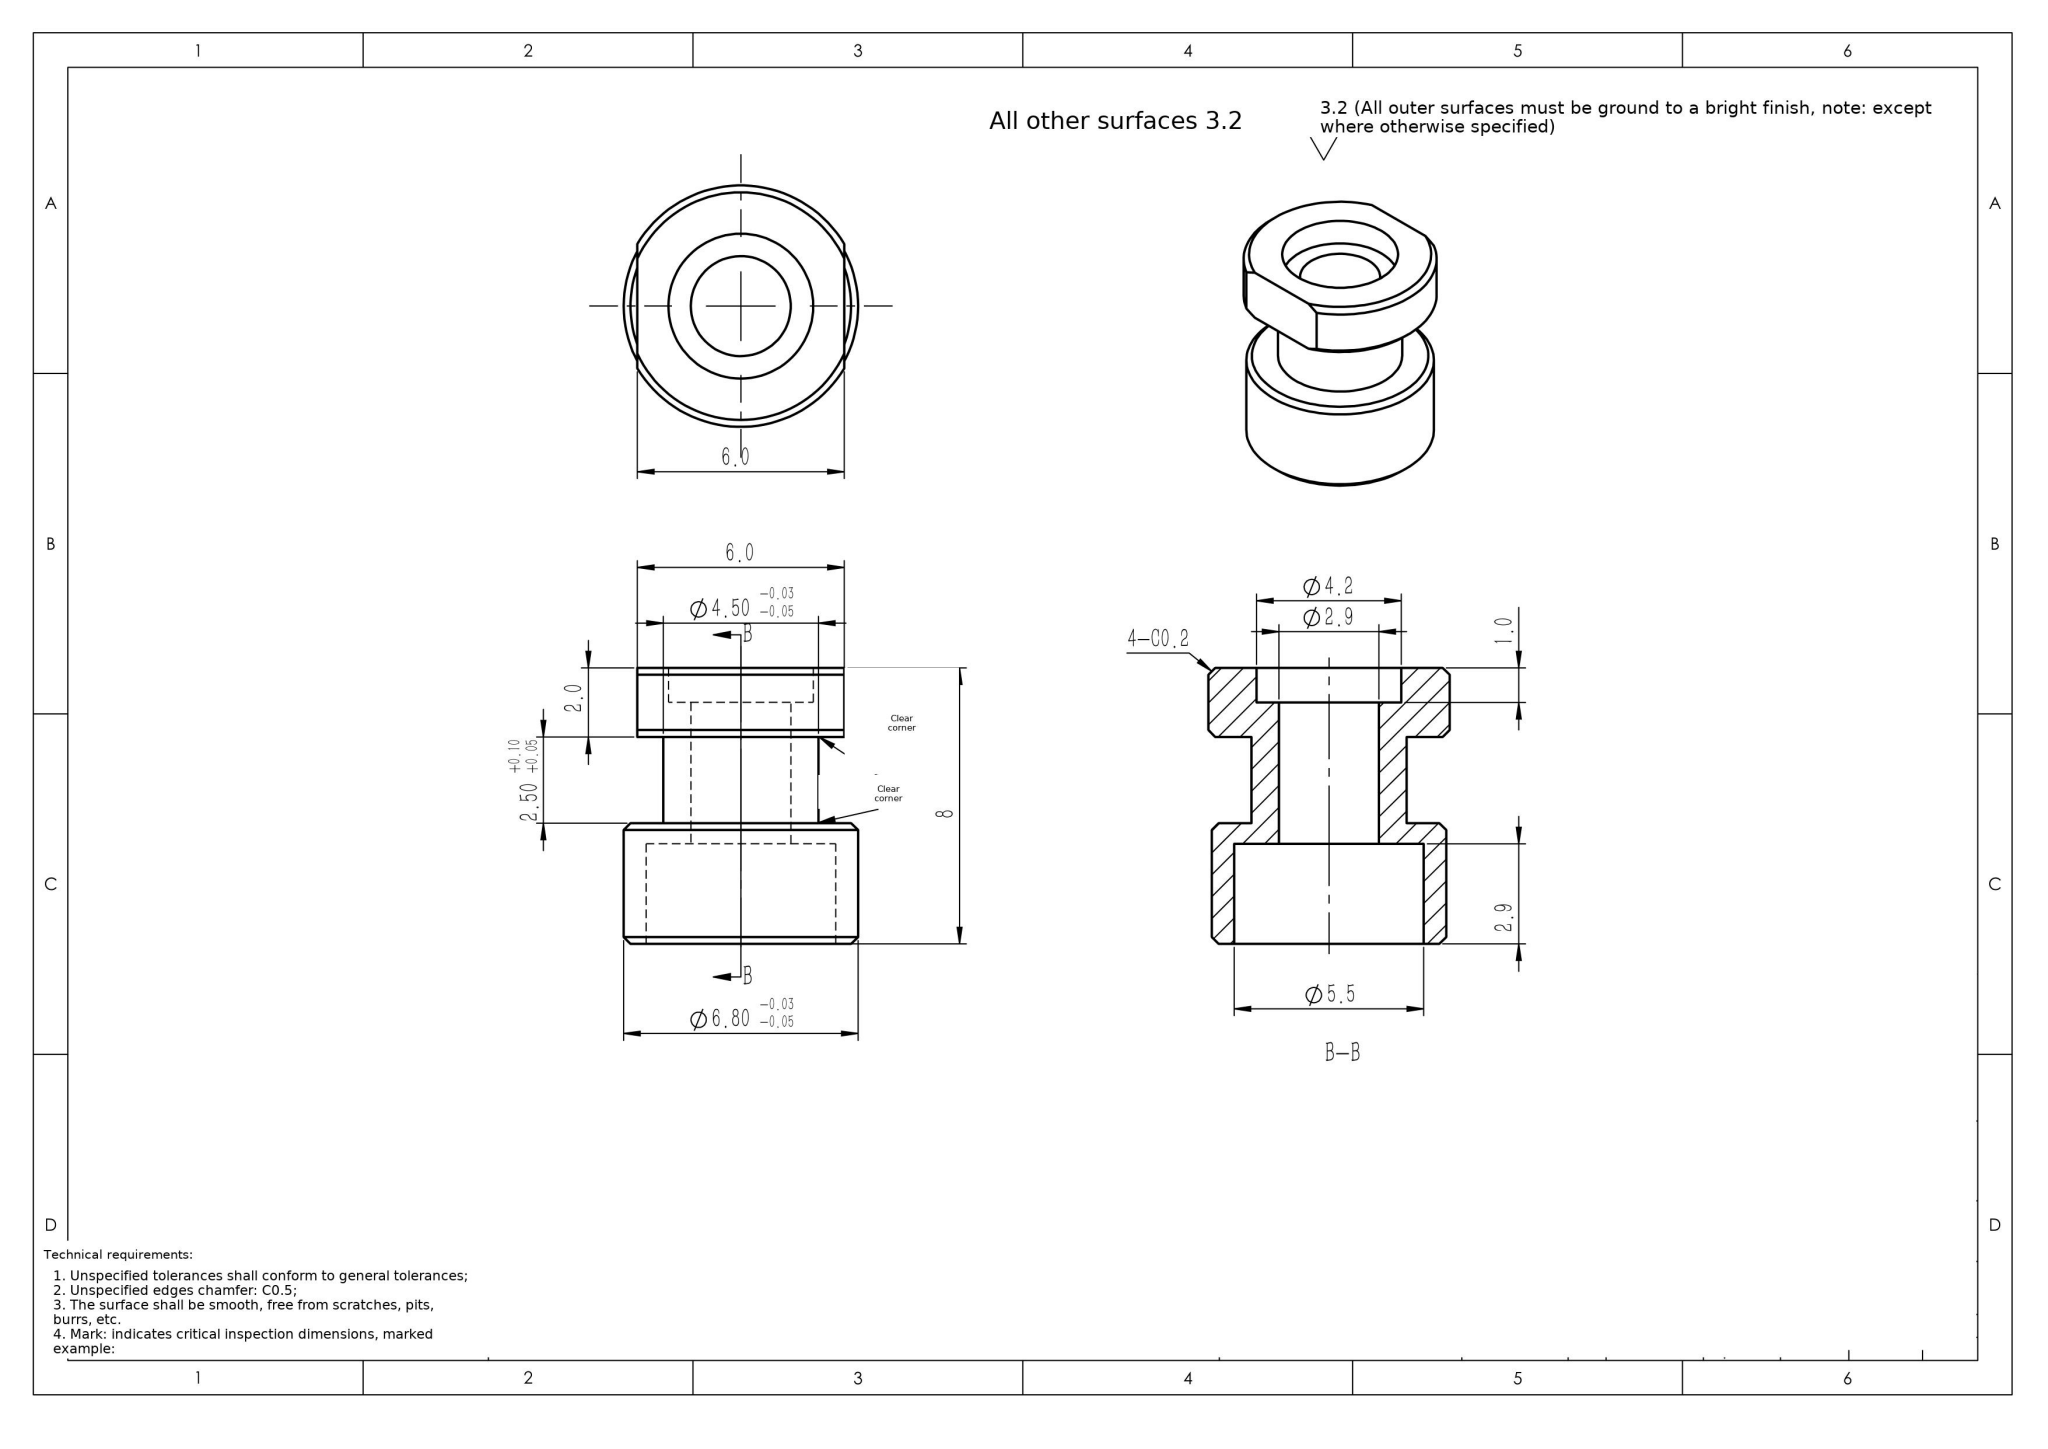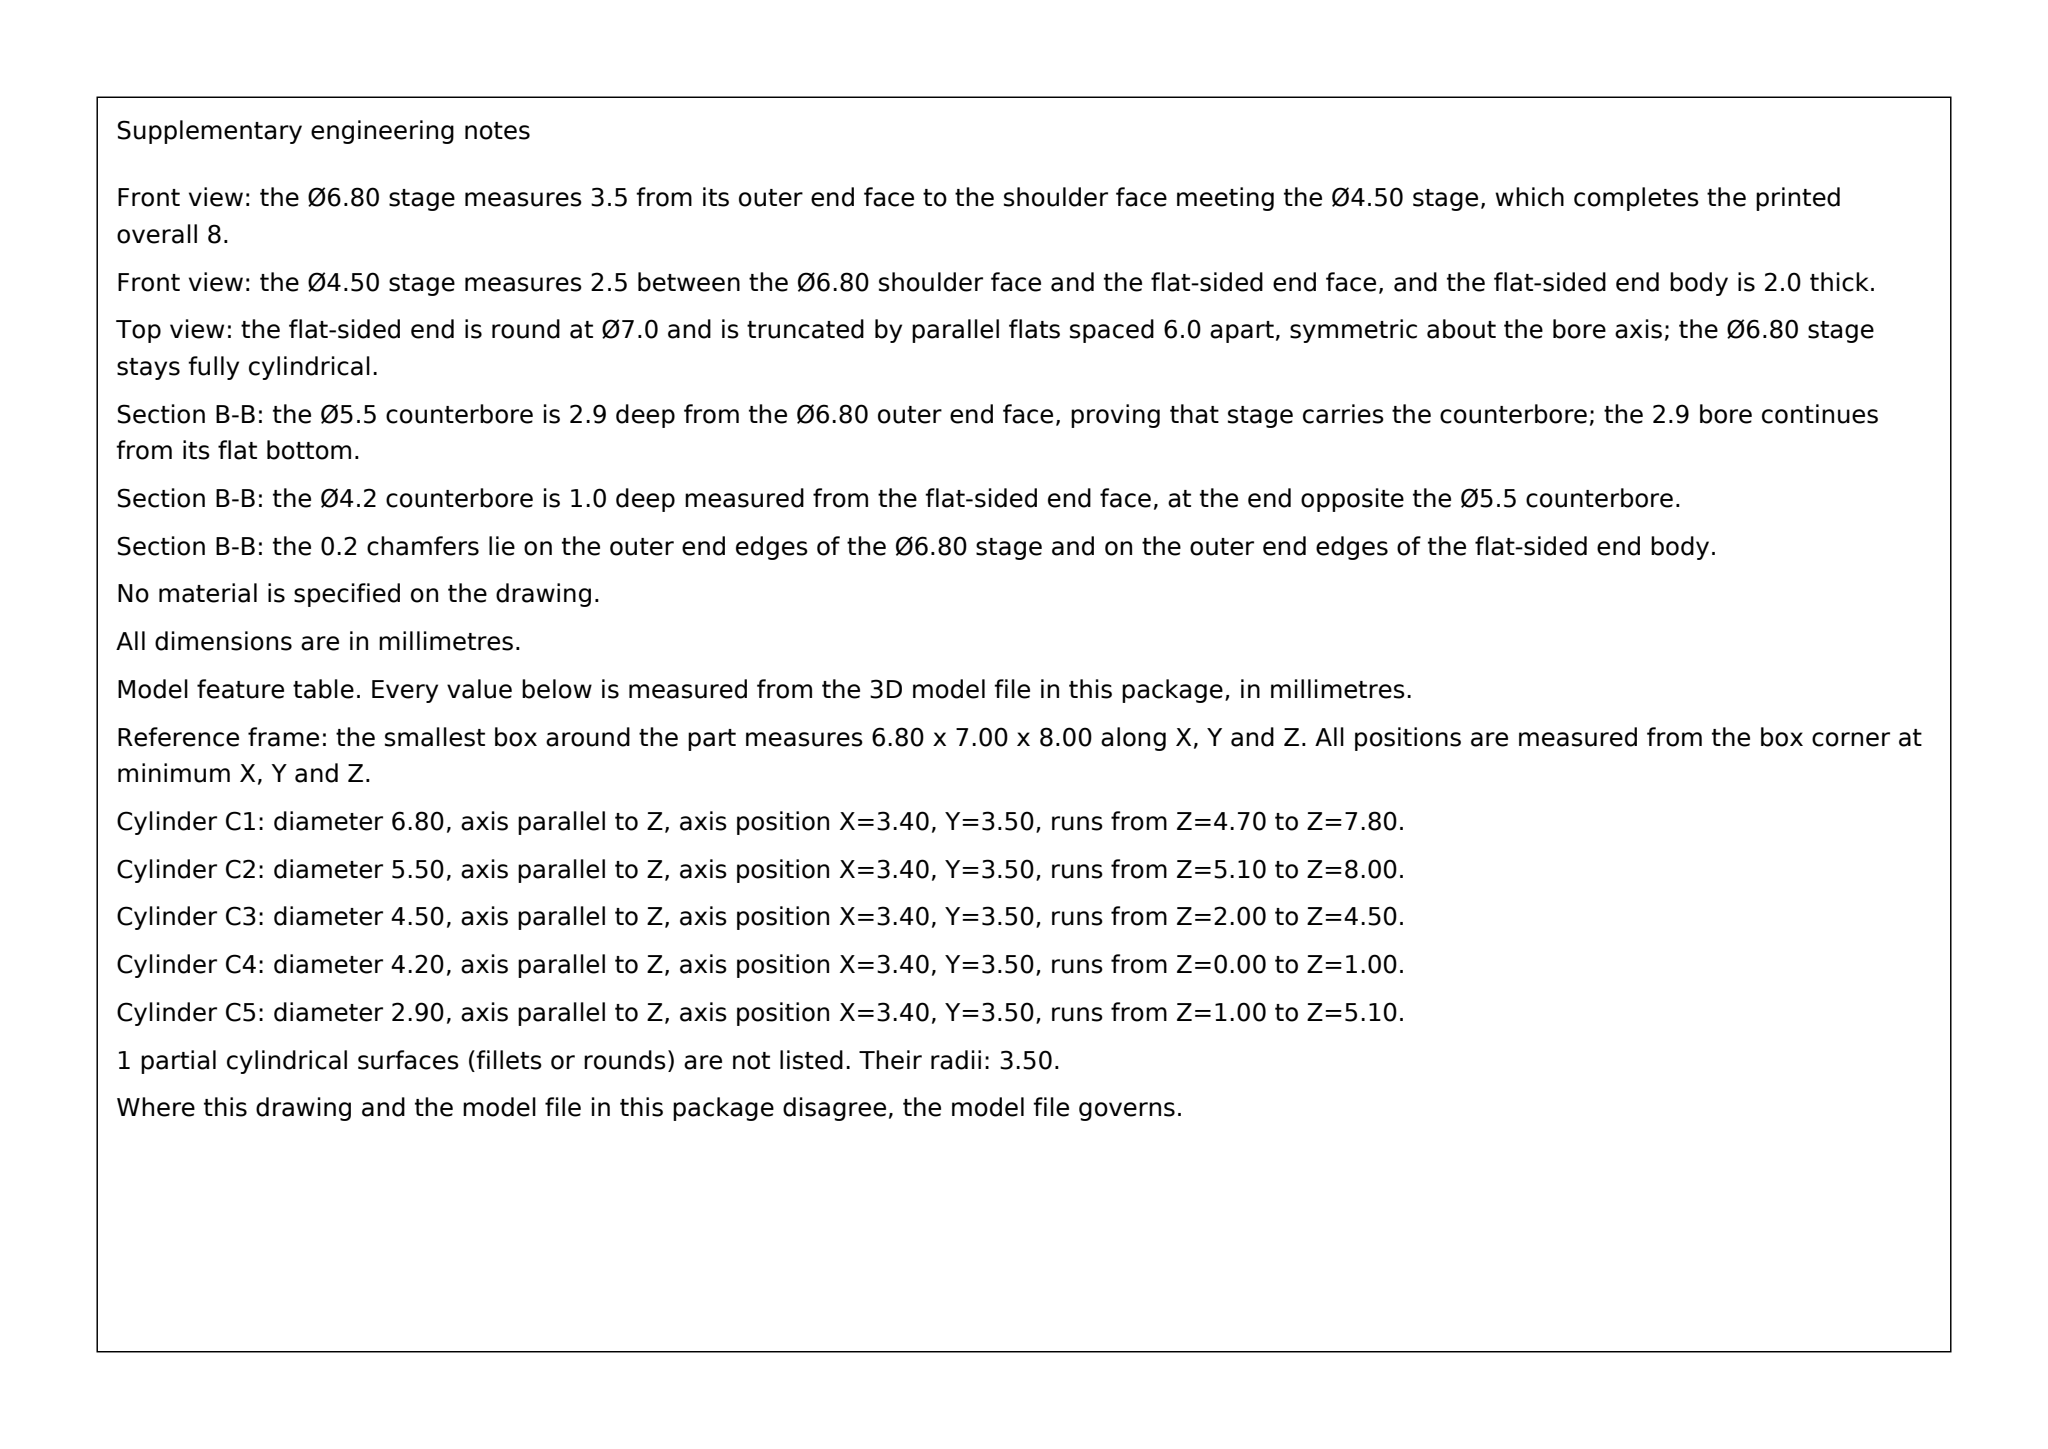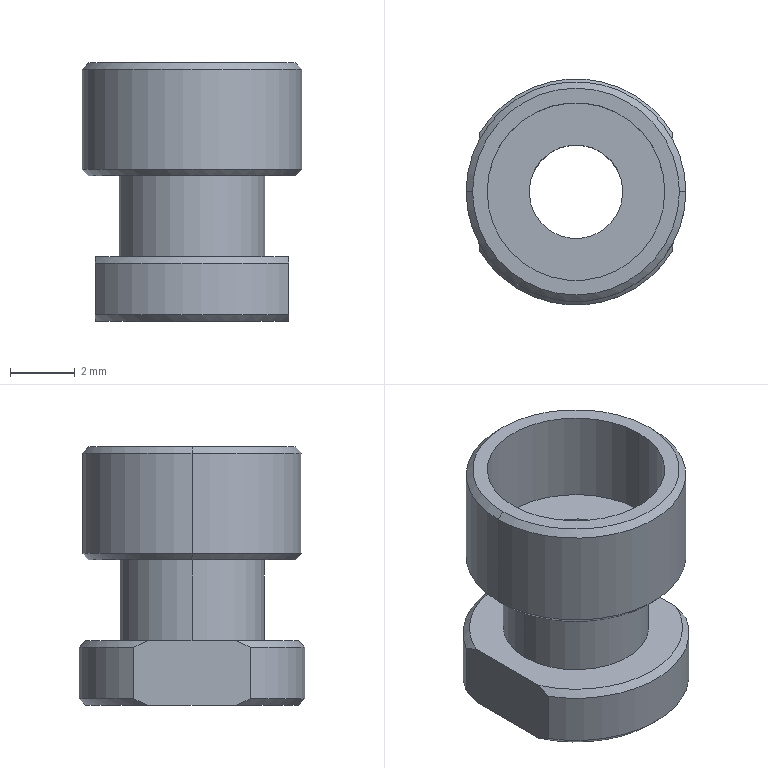Part | SolidWorks | mm | 1 solid | 28 faces | box 6.8 x 7 x 8 mm | volume 128 mm3 | cylinder 12 | cone 8 | plane 8 | commonest cylinder face diameters 4.2 x2 5.5 x2 4.5 x2 6.8 x2 2.9 x2 7 x2
Drawing notes:
Ø7.0 FLANGE W/ 2 FLATS 6.0 APART, 2.0 THK - NOT Ø6.80 BOSS | from the solid: Convex arc dia 7.0, axis z, z 0.2-1.8, arc 236 deg, with planes x=0.4 and x=6.4 (6.0 across flats), flange z 0.0-2.0; separate boss/shaft dia 6.8 z 4.7-7.8
build123d program:
from build123d import *

# Parameters (mm, degrees)
SKETCH1_R                                         = 3.4
BOSS_EXTRUDE1_DEPTH                               = 3.5
SKETCH2_R                                         = 2.25
BOSS_EXTRUDE2_DEPTH                               = 2.5
SKETCH3_R                                         = 3.5
BOSS_EXTRUDE3_DEPTH                               = 2
M2_5_HEX_SOCKET_HEAD_CAP_SCREW_CBORE2_D           = 2.9
M2_5_HEX_SOCKET_HEAD_CAP_SCREW_CBORE2_DEPTH       = 11.5
M2_5_HEX_SOCKET_HEAD_CAP_SCREW_CBORE2_CBORE_D     = 5.5
M2_5_HEX_SOCKET_HEAD_CAP_SCREW_CBORE2_CBORE_DEPTH = 2.9
M2_5_HEX_SOCKET_HEAD_CAP_SCREW_CBORE2_TIP         = 0.8712
SKETCH8_R                                         = 2.1
CUT_EXTRUDE1_DEPTH                                = 1
SKETCH9_W                                         = 1
SKETCH9_H                                         = 3.606
CUT_EXTRUDE2_DEPTH                                = 2
CHAMFER1_SIZE                                     = 0.2


with BuildPart() as part:
    # Sketch1 → Boss-Extrude1 (new body)
    with BuildSketch(Plane.XY):
        Circle(SKETCH1_R)
    extrude(amount=BOSS_EXTRUDE1_DEPTH)

    # Sketch2 → Boss-Extrude2 (add)
    with BuildSketch(Plane(origin=(0, 0, 0), x_dir=(-1, 0, 0), z_dir=(0, 0, -1))):
        with Locations(Location((0, 0, 0), (0, 0, 180))):
            Circle(SKETCH2_R)
    extrude(amount=BOSS_EXTRUDE2_DEPTH)

    # Sketch3 → Boss-Extrude3 (add)
    with BuildSketch(Plane(origin=(0, 0, -2.5), x_dir=(-1, 0, 0), z_dir=(0, 0, -1))):
        Circle(SKETCH3_R)
    extrude(amount=BOSS_EXTRUDE3_DEPTH)

    # M2.5 Hex Socket Head Cap Screw CBORE2
    with Locations(Plane.XY.offset(3.5)):
        with Locations((0, 0)):
            CounterBoreHole(M2_5_HEX_SOCKET_HEAD_CAP_SCREW_CBORE2_D / 2, M2_5_HEX_SOCKET_HEAD_CAP_SCREW_CBORE2_CBORE_D / 2, M2_5_HEX_SOCKET_HEAD_CAP_SCREW_CBORE2_CBORE_DEPTH, depth=M2_5_HEX_SOCKET_HEAD_CAP_SCREW_CBORE2_DEPTH)
            with Locations((0, 0, -(M2_5_HEX_SOCKET_HEAD_CAP_SCREW_CBORE2_DEPTH + M2_5_HEX_SOCKET_HEAD_CAP_SCREW_CBORE2_TIP / 2))):  # 118° drill point
                Cone(0, M2_5_HEX_SOCKET_HEAD_CAP_SCREW_CBORE2_D / 2, M2_5_HEX_SOCKET_HEAD_CAP_SCREW_CBORE2_TIP, mode=Mode.SUBTRACT)

    # Sketch8 → Cut-Extrude1 (cut)
    with BuildSketch(Plane(origin=(0, 0, -4.5), x_dir=(-1, 0, 0), z_dir=(0, 0, -1))):
        Circle(SKETCH8_R)
    extrude(amount=-CUT_EXTRUDE1_DEPTH, mode=Mode.SUBTRACT)

    # Sketch9 → Cut-Extrude2 (cut)
    with BuildSketch(Plane(origin=(0, 0, -4.5), x_dir=(-1, 0, 0), z_dir=(0, 0, -1))):
        with Locations((3.5, 0)):
            Rectangle(SKETCH9_W, SKETCH9_H)
        with Locations((-3.5, 0)):
            Rectangle(SKETCH9_W, SKETCH9_H)
    extrude(amount=-CUT_EXTRUDE2_DEPTH, mode=Mode.SUBTRACT)

    # Chamfer1
    chamfer1_edges = [part.edges().sort_by_distance(p)[0] for p in [
        (-3.4, 0, 0),
        (-3.4, 0, 3.5),
        (0, -3.5, -2.5),
        (0, -3.5, -4.5),
        (0, 3.5, -2.5),
        (0, 3.5, -4.5),
    ]]
    chamfer(chamfer1_edges, length=CHAMFER1_SIZE)


solid = part.part
STEP:
#1=CARTESIAN_POINT('',(3.2,0.,3.5));
#2=VERTEX_POINT('',#1);
#3=CARTESIAN_POINT('',(-3.2,0.,3.5));
#4=VERTEX_POINT('',#3);
#5=CARTESIAN_POINT('',(0.,0.,3.5));
#6=DIRECTION('',(0.,0.,1.));
#7=DIRECTION('',(1.,0.,0.));
#8=AXIS2_PLACEMENT_3D('',#5,#6,#7);
#9=CIRCLE('',#8,3.2);
#10=EDGE_CURVE('',#2,#4,#9,.T.);
#11=ORIENTED_EDGE('',*,*,#10,.F.);
#12=CARTESIAN_POINT('',(3.4,0.,3.3));
#13=VERTEX_POINT('',#12);
#14=CARTESIAN_POINT('',(3.2,0.,3.5));
#15=DIRECTION('',(0.7071,0.,-0.7071));
#16=VECTOR('',#15,1000.);
#17=LINE('',#14,#16);
#18=EDGE_CURVE('',#2,#13,#17,.T.);
#19=ORIENTED_EDGE('',*,*,#18,.T.);
#20=CARTESIAN_POINT('',(-3.4,0.,3.3));
#21=VERTEX_POINT('',#20);
#22=CARTESIAN_POINT('',(0.,0.,3.3));
#23=DIRECTION('',(0.,0.,-1.));
#24=DIRECTION('',(1.,0.,0.));
#25=AXIS2_PLACEMENT_3D('',#22,#23,#24);
#26=CIRCLE('',#25,3.4);
#27=EDGE_CURVE('',#21,#13,#26,.T.);
#28=ORIENTED_EDGE('',*,*,#27,.F.);
#29=CARTESIAN_POINT('',(-3.2,0.,3.5));
#30=DIRECTION('',(-0.7071,0.,-0.7071));
#31=VECTOR('',#30,1000.);
#32=LINE('',#29,#31);
#33=EDGE_CURVE('',#4,#21,#32,.T.);
#34=ORIENTED_EDGE('',*,*,#33,.F.);
#35=EDGE_LOOP('',(#11,#19,#28,#34));
#36=FACE_OUTER_BOUND('',#35,.T.);
#37=CARTESIAN_POINT('',(0.,0.,3.5));
#38=DIRECTION('',(0.,0.,-1.));
#39=DIRECTION('',(-1.,0.,0.));
#40=AXIS2_PLACEMENT_3D('',#37,#38,#39);
#41=CONICAL_SURFACE('',#40,3.2,0.7854);
#42=ADVANCED_FACE('',(#36),#41,.T.);
#43=CARTESIAN_POINT('',(-3.2,0.,0.));
#44=VERTEX_POINT('',#43);
#45=CARTESIAN_POINT('',(3.2,0.,0.));
#46=VERTEX_POINT('',#45);
#47=CARTESIAN_POINT('',(0.,0.,0.));
#48=DIRECTION('',(0.,0.,-1.));
#49=DIRECTION('',(1.,0.,0.));
#50=AXIS2_PLACEMENT_3D('',#47,#48,#49);
#51=CIRCLE('',#50,3.2);
#52=EDGE_CURVE('',#44,#46,#51,.T.);
#53=ORIENTED_EDGE('',*,*,#52,.F.);
#54=CARTESIAN_POINT('',(-3.4,0.,0.2));
#55=VERTEX_POINT('',#54);
#56=CARTESIAN_POINT('',(-3.4,0.,0.2));
#57=DIRECTION('',(-0.7071,0.,0.7071));
#58=VECTOR('',#57,1000.);
#59=LINE('',#56,#58);
#60=EDGE_CURVE('',#44,#55,#59,.T.);
#61=ORIENTED_EDGE('',*,*,#60,.T.);
#62=CARTESIAN_POINT('',(3.4,0.,0.2));
#63=VERTEX_POINT('',#62);
#64=CARTESIAN_POINT('',(0.,0.,0.2));
#65=DIRECTION('',(0.,0.,1.));
#66=DIRECTION('',(1.,0.,0.));
#67=AXIS2_PLACEMENT_3D('',#64,#65,#66);
#68=CIRCLE('',#67,3.4);
#69=EDGE_CURVE('',#63,#55,#68,.T.);
#70=ORIENTED_EDGE('',*,*,#69,.F.);
#71=CARTESIAN_POINT('',(3.4,0.,0.2));
#72=DIRECTION('',(0.7071,0.,0.7071));
#73=VECTOR('',#72,1000.);
#74=LINE('',#71,#73);
#75=EDGE_CURVE('',#46,#63,#74,.T.);
#76=ORIENTED_EDGE('',*,*,#75,.F.);
#77=EDGE_LOOP('',(#53,#61,#70,#76));
#78=FACE_OUTER_BOUND('',#77,.T.);
#79=CARTESIAN_POINT('',(0.,0.,0.2));
#80=DIRECTION('',(0.,0.,1.));
#81=DIRECTION('',(1.,0.,0.));
#82=AXIS2_PLACEMENT_3D('',#79,#80,#81);
#83=CONICAL_SURFACE('',#82,3.4,0.7854);
#84=ADVANCED_FACE('',(#78),#83,.T.);
#85=CARTESIAN_POINT('',(2.1,0.,-3.5));
#86=VERTEX_POINT('',#85);
#87=CARTESIAN_POINT('',(-2.1,0.,-3.5));
#88=VERTEX_POINT('',#87);
#89=CARTESIAN_POINT('',(0.,0.,-3.5));
#90=DIRECTION('',(0.,0.,-1.));
#91=DIRECTION('',(-1.,0.,0.));
#92=AXIS2_PLACEMENT_3D('',#89,#90,#91);
#93=CIRCLE('',#92,2.1);
#94=EDGE_CURVE('',#86,#88,#93,.T.);
#95=ORIENTED_EDGE('',*,*,#94,.F.);
#96=CARTESIAN_POINT('',(2.1,0.,-4.5));
#97=VERTEX_POINT('',#96);
#98=CARTESIAN_POINT('',(2.1,0.,-3.5));
#99=DIRECTION('',(0.,0.,-1.));
#100=VECTOR('',#99,1000.);
#101=LINE('',#98,#100);
#102=EDGE_CURVE('',#86,#97,#101,.T.);
#103=ORIENTED_EDGE('',*,*,#102,.T.);
#104=CARTESIAN_POINT('',(-2.1,0.,-4.5));
#105=VERTEX_POINT('',#104);
#106=CARTESIAN_POINT('',(0.,0.,-4.5));
#107=DIRECTION('',(0.,0.,-1.));
#108=DIRECTION('',(-1.,0.,0.));
#109=AXIS2_PLACEMENT_3D('',#106,#107,#108);
#110=CIRCLE('',#109,2.1);
#111=EDGE_CURVE('',#97,#105,#110,.T.);
#112=ORIENTED_EDGE('',*,*,#111,.T.);
#113=CARTESIAN_POINT('',(-2.1,0.,-3.5));
#114=DIRECTION('',(0.,0.,-1.));
#115=VECTOR('',#114,1000.);
#116=LINE('',#113,#115);
#117=EDGE_CURVE('',#88,#105,#116,.T.);
#118=ORIENTED_EDGE('',*,*,#117,.F.);
#119=EDGE_LOOP('',(#95,#103,#112,#118));
#120=FACE_OUTER_BOUND('',#119,.T.);
#121=CARTESIAN_POINT('',(0.,0.,-3.5));
#122=DIRECTION('',(0.,0.,-1.));
#123=DIRECTION('',(-1.,0.,0.));
#124=AXIS2_PLACEMENT_3D('',#121,#122,#123);
#125=CYLINDRICAL_SURFACE('',#124,2.1);
#126=ADVANCED_FACE('',(#120),#125,.F.);
#127=CARTESIAN_POINT('',(-2.75,0.,0.6));
#128=VERTEX_POINT('',#127);
#129=CARTESIAN_POINT('',(2.75,0.,0.6));
#130=VERTEX_POINT('',#129);
#131=CARTESIAN_POINT('',(0.,0.,0.6));
#132=DIRECTION('',(0.,0.,1.));
#133=DIRECTION('',(1.,0.,0.));
#134=AXIS2_PLACEMENT_3D('',#131,#132,#133);
#135=CIRCLE('',#134,2.75);
#136=EDGE_CURVE('',#128,#130,#135,.T.);
#137=ORIENTED_EDGE('',*,*,#136,.F.);
#138=CARTESIAN_POINT('',(-2.75,0.,3.5));
#139=VERTEX_POINT('',#138);
#140=CARTESIAN_POINT('',(-2.75,0.,3.5));
#141=DIRECTION('',(0.,0.,1.));
#142=VECTOR('',#141,1000.);
#143=LINE('',#140,#142);
#144=EDGE_CURVE('',#128,#139,#143,.T.);
#145=ORIENTED_EDGE('',*,*,#144,.T.);
#146=CARTESIAN_POINT('',(2.75,0.,3.5));
#147=VERTEX_POINT('',#146);
#148=CARTESIAN_POINT('',(0.,0.,3.5));
#149=DIRECTION('',(0.,0.,1.));
#150=DIRECTION('',(1.,0.,0.));
#151=AXIS2_PLACEMENT_3D('',#148,#149,#150);
#152=CIRCLE('',#151,2.75);
#153=EDGE_CURVE('',#139,#147,#152,.T.);
#154=ORIENTED_EDGE('',*,*,#153,.T.);
#155=CARTESIAN_POINT('',(2.75,0.,3.5));
#156=DIRECTION('',(0.,0.,1.));
#157=VECTOR('',#156,1000.);
#158=LINE('',#155,#157);
#159=EDGE_CURVE('',#130,#147,#158,.T.);
#160=ORIENTED_EDGE('',*,*,#159,.F.);
#161=EDGE_LOOP('',(#137,#145,#154,#160));
#162=FACE_OUTER_BOUND('',#161,.T.);
#163=CARTESIAN_POINT('',(0.,0.,3.5));
#164=DIRECTION('',(0.,0.,1.));
#165=DIRECTION('',(1.,0.,0.));
#166=AXIS2_PLACEMENT_3D('',#163,#164,#165);
#167=CYLINDRICAL_SURFACE('',#166,2.75);
#168=ADVANCED_FACE('',(#162),#167,.F.);
#169=CARTESIAN_POINT('',(-2.25,0.,-2.5));
#170=VERTEX_POINT('',#169);
#171=CARTESIAN_POINT('',(2.25,0.,-2.5));
#172=VERTEX_POINT('',#171);
#173=CARTESIAN_POINT('',(0.,0.,-2.5));
#174=DIRECTION('',(0.,0.,-1.));
#175=DIRECTION('',(-1.,0.,0.));
#176=AXIS2_PLACEMENT_3D('',#173,#174,#175);
#177=CIRCLE('',#176,2.25);
#178=EDGE_CURVE('',#170,#172,#177,.T.);
#179=ORIENTED_EDGE('',*,*,#178,.F.);
#180=CARTESIAN_POINT('',(-2.25,0.,0.));
#181=VERTEX_POINT('',#180);
#182=CARTESIAN_POINT('',(-2.25,0.,-2.5));
#183=DIRECTION('',(0.,0.,1.));
#184=VECTOR('',#183,1000.);
#185=LINE('',#182,#184);
#186=EDGE_CURVE('',#170,#181,#185,.T.);
#187=ORIENTED_EDGE('',*,*,#186,.T.);
#188=CARTESIAN_POINT('',(2.25,0.,0.));
#189=VERTEX_POINT('',#188);
#190=CARTESIAN_POINT('',(0.,0.,0.));
#191=DIRECTION('',(0.,0.,-1.));
#192=DIRECTION('',(1.,0.,0.));
#193=AXIS2_PLACEMENT_3D('',#190,#191,#192);
#194=CIRCLE('',#193,2.25);
#195=EDGE_CURVE('',#181,#189,#194,.T.);
#196=ORIENTED_EDGE('',*,*,#195,.T.);
#197=CARTESIAN_POINT('',(2.25,0.,-2.5));
#198=DIRECTION('',(0.,0.,1.));
#199=VECTOR('',#198,1000.);
#200=LINE('',#197,#199);
#201=EDGE_CURVE('',#172,#189,#200,.T.);
#202=ORIENTED_EDGE('',*,*,#201,.F.);
#203=EDGE_LOOP('',(#179,#187,#196,#202));
#204=FACE_OUTER_BOUND('',#203,.T.);
#205=CARTESIAN_POINT('',(0.,0.,-2.5));
#206=DIRECTION('',(0.,0.,1.));
#207=DIRECTION('',(1.,0.,0.));
#208=AXIS2_PLACEMENT_3D('',#205,#206,#207);
#209=CYLINDRICAL_SURFACE('',#208,2.25);
#210=ADVANCED_FACE('',(#204),#209,.T.);
#211=ORIENTED_EDGE('',*,*,#27,.T.);
#212=CARTESIAN_POINT('',(3.4,0.,3.5));
#213=DIRECTION('',(0.,0.,-1.));
#214=VECTOR('',#213,1000.);
#215=LINE('',#212,#214);
#216=EDGE_CURVE('',#13,#63,#215,.T.);
#217=ORIENTED_EDGE('',*,*,#216,.T.);
#218=ORIENTED_EDGE('',*,*,#69,.T.);
#219=CARTESIAN_POINT('',(-3.4,0.,3.5));
#220=DIRECTION('',(0.,0.,-1.));
#221=VECTOR('',#220,1000.);
#222=LINE('',#219,#221);
#223=EDGE_CURVE('',#21,#55,#222,.T.);
#224=ORIENTED_EDGE('',*,*,#223,.F.);
#225=EDGE_LOOP('',(#211,#217,#218,#224));
#226=FACE_OUTER_BOUND('',#225,.T.);
#227=CARTESIAN_POINT('',(0.,0.,3.5));
#228=DIRECTION('',(0.,0.,-1.));
#229=DIRECTION('',(-1.,0.,0.));
#230=AXIS2_PLACEMENT_3D('',#227,#228,#229);
#231=CYLINDRICAL_SURFACE('',#230,3.4);
#232=ADVANCED_FACE('',(#226),#231,.T.);
#233=CARTESIAN_POINT('',(-1.45,0.,-3.5));
#234=VERTEX_POINT('',#233);
#235=CARTESIAN_POINT('',(1.45,0.,-3.5));
#236=VERTEX_POINT('',#235);
#237=CARTESIAN_POINT('',(0.,0.,-3.5));
#238=DIRECTION('',(0.,0.,1.));
#239=DIRECTION('',(-1.,0.,0.));
#240=AXIS2_PLACEMENT_3D('',#237,#238,#239);
#241=CIRCLE('',#240,1.45);
#242=EDGE_CURVE('',#234,#236,#241,.T.);
#243=ORIENTED_EDGE('',*,*,#242,.F.);
#244=CARTESIAN_POINT('',(-1.45,0.,0.6));
#245=VERTEX_POINT('',#244);
#246=CARTESIAN_POINT('',(-1.45,0.,3.5));
#247=DIRECTION('',(0.,0.,1.));
#248=VECTOR('',#247,1000.);
#249=LINE('',#246,#248);
#250=EDGE_CURVE('',#234,#245,#249,.T.);
#251=ORIENTED_EDGE('',*,*,#250,.T.);
#252=CARTESIAN_POINT('',(1.45,0.,0.6));
#253=VERTEX_POINT('',#252);
#254=CARTESIAN_POINT('',(0.,0.,0.6));
#255=DIRECTION('',(0.,0.,1.));
#256=DIRECTION('',(1.,0.,0.));
#257=AXIS2_PLACEMENT_3D('',#254,#255,#256);
#258=CIRCLE('',#257,1.45);
#259=EDGE_CURVE('',#245,#253,#258,.T.);
#260=ORIENTED_EDGE('',*,*,#259,.T.);
#261=CARTESIAN_POINT('',(1.45,0.,3.5));
#262=DIRECTION('',(0.,0.,1.));
#263=VECTOR('',#262,1000.);
#264=LINE('',#261,#263);
#265=EDGE_CURVE('',#236,#253,#264,.T.);
#266=ORIENTED_EDGE('',*,*,#265,.F.);
#267=EDGE_LOOP('',(#243,#251,#260,#266));
#268=FACE_OUTER_BOUND('',#267,.T.);
#269=CARTESIAN_POINT('',(0.,0.,3.5));
#270=DIRECTION('',(0.,0.,1.));
#271=DIRECTION('',(1.,0.,0.));
#272=AXIS2_PLACEMENT_3D('',#269,#270,#271);
#273=CYLINDRICAL_SURFACE('',#272,1.45);
#274=ADVANCED_FACE('',(#268),#273,.F.);
#275=CARTESIAN_POINT('',(-3.,-1.803,-2.7));
#276=VERTEX_POINT('',#275);
#277=CARTESIAN_POINT('',(-3.,-1.803,-4.3));
#278=VERTEX_POINT('',#277);
#279=CARTESIAN_POINT('',(-3.,-1.803,1.242));
#280=DIRECTION('',(0.,0.,-1.));
#281=VECTOR('',#280,1000.);
#282=LINE('',#279,#281);
#283=EDGE_CURVE('',#276,#278,#282,.T.);
#284=ORIENTED_EDGE('',*,*,#283,.T.);
#285=CARTESIAN_POINT('',(3.,-1.803,-4.3));
#286=VERTEX_POINT('',#285);
#287=CARTESIAN_POINT('',(0.,0.,-4.3));
#288=DIRECTION('',(0.,0.,1.));
#289=DIRECTION('',(-1.,0.,0.));
#290=AXIS2_PLACEMENT_3D('',#287,#288,#289);
#291=CIRCLE('',#290,3.5);
#292=EDGE_CURVE('',#278,#286,#291,.T.);
#293=ORIENTED_EDGE('',*,*,#292,.T.);
#294=CARTESIAN_POINT('',(3.,-1.803,-2.7));
#295=VERTEX_POINT('',#294);
#296=CARTESIAN_POINT('',(3.,-1.803,1.242));
#297=DIRECTION('',(0.,0.,-1.));
#298=VECTOR('',#297,1000.);
#299=LINE('',#296,#298);
#300=EDGE_CURVE('',#295,#286,#299,.T.);
#301=ORIENTED_EDGE('',*,*,#300,.F.);
#302=CARTESIAN_POINT('',(0.,0.,-2.7));
#303=DIRECTION('',(0.,0.,-1.));
#304=DIRECTION('',(-1.,0.,0.));
#305=AXIS2_PLACEMENT_3D('',#302,#303,#304);
#306=CIRCLE('',#305,3.5);
#307=EDGE_CURVE('',#295,#276,#306,.T.);
#308=ORIENTED_EDGE('',*,*,#307,.T.);
#309=EDGE_LOOP('',(#284,#293,#301,#308));
#310=FACE_OUTER_BOUND('',#309,.T.);
#311=CARTESIAN_POINT('',(0.,0.,-4.5));
#312=DIRECTION('',(0.,0.,1.));
#313=DIRECTION('',(1.,0.,0.));
#314=AXIS2_PLACEMENT_3D('',#311,#312,#313);
#315=CYLINDRICAL_SURFACE('',#314,3.5);
#316=ADVANCED_FACE('',(#310),#315,.T.);
#317=ORIENTED_EDGE('',*,*,#250,.F.);
#318=CARTESIAN_POINT('',(0.,0.,-3.5));
#319=DIRECTION('',(0.,0.,1.));
#320=DIRECTION('',(-1.,0.,0.));
#321=AXIS2_PLACEMENT_3D('',#318,#319,#320);
#322=CIRCLE('',#321,1.45);
#323=EDGE_CURVE('',#236,#234,#322,.T.);
#324=ORIENTED_EDGE('',*,*,#323,.F.);
#325=ORIENTED_EDGE('',*,*,#265,.T.);
#326=CARTESIAN_POINT('',(0.,0.,0.6));
#327=DIRECTION('',(0.,0.,1.));
#328=DIRECTION('',(1.,0.,0.));
#329=AXIS2_PLACEMENT_3D('',#326,#327,#328);
#330=CIRCLE('',#329,1.45);
#331=EDGE_CURVE('',#253,#245,#330,.T.);
#332=ORIENTED_EDGE('',*,*,#331,.T.);
#333=EDGE_LOOP('',(#317,#324,#325,#332));
#334=FACE_OUTER_BOUND('',#333,.T.);
#335=CARTESIAN_POINT('',(0.,0.,3.5));
#336=DIRECTION('',(0.,0.,1.));
#337=DIRECTION('',(1.,0.,0.));
#338=AXIS2_PLACEMENT_3D('',#335,#336,#337);
#339=CYLINDRICAL_SURFACE('',#338,1.45);
#340=ADVANCED_FACE('',(#334),#339,.F.);
#341=ORIENTED_EDGE('',*,*,#216,.F.);
#342=CARTESIAN_POINT('',(0.,0.,3.3));
#343=DIRECTION('',(0.,0.,-1.));
#344=DIRECTION('',(1.,0.,0.));
#345=AXIS2_PLACEMENT_3D('',#342,#343,#344);
#346=CIRCLE('',#345,3.4);
#347=EDGE_CURVE('',#13,#21,#346,.T.);
#348=ORIENTED_EDGE('',*,*,#347,.T.);
#349=ORIENTED_EDGE('',*,*,#223,.T.);
#350=CARTESIAN_POINT('',(0.,0.,0.2));
#351=DIRECTION('',(0.,0.,1.));
#352=DIRECTION('',(1.,0.,0.));
#353=AXIS2_PLACEMENT_3D('',#350,#351,#352);
#354=CIRCLE('',#353,3.4);
#355=EDGE_CURVE('',#55,#63,#354,.T.);
#356=ORIENTED_EDGE('',*,*,#355,.T.);
#357=EDGE_LOOP('',(#341,#348,#349,#356));
#358=FACE_OUTER_BOUND('',#357,.T.);
#359=CARTESIAN_POINT('',(0.,0.,3.5));
#360=DIRECTION('',(0.,0.,-1.));
#361=DIRECTION('',(-1.,0.,0.));
#362=AXIS2_PLACEMENT_3D('',#359,#360,#361);
#363=CYLINDRICAL_SURFACE('',#362,3.4);
#364=ADVANCED_FACE('',(#358),#363,.T.);
#365=CARTESIAN_POINT('',(0.,0.,3.5));
#366=DIRECTION('',(0.,0.,1.));
#367=DIRECTION('',(1.,0.,0.));
#368=AXIS2_PLACEMENT_3D('',#365,#366,#367);
#369=CIRCLE('',#368,3.2);
#370=EDGE_CURVE('',#4,#2,#369,.T.);
#371=ORIENTED_EDGE('',*,*,#370,.T.);
#372=ORIENTED_EDGE('',*,*,#10,.T.);
#373=EDGE_LOOP('',(#371,#372));
#374=FACE_OUTER_BOUND('',#373,.T.);
#375=CARTESIAN_POINT('',(0.,0.,3.5));
#376=DIRECTION('',(0.,0.,1.));
#377=DIRECTION('',(1.,0.,0.));
#378=AXIS2_PLACEMENT_3D('',#375,#376,#377);
#379=CIRCLE('',#378,2.75);
#380=EDGE_CURVE('',#147,#139,#379,.T.);
#381=ORIENTED_EDGE('',*,*,#380,.F.);
#382=ORIENTED_EDGE('',*,*,#153,.F.);
#383=EDGE_LOOP('',(#381,#382));
#384=FACE_BOUND('',#383,.T.);
#385=CARTESIAN_POINT('',(0.,0.,3.5));
#386=DIRECTION('',(0.,0.,1.));
#387=DIRECTION('',(1.,0.,0.));
#388=AXIS2_PLACEMENT_3D('',#385,#386,#387);
#389=PLANE('',#388);
#390=ADVANCED_FACE('',(#374,#384),#389,.T.);
#391=CARTESIAN_POINT('',(0.,0.,0.));
#392=DIRECTION('',(0.,0.,-1.));
#393=DIRECTION('',(1.,0.,0.));
#394=AXIS2_PLACEMENT_3D('',#391,#392,#393);
#395=CIRCLE('',#394,3.2);
#396=EDGE_CURVE('',#46,#44,#395,.T.);
#397=ORIENTED_EDGE('',*,*,#396,.T.);
#398=ORIENTED_EDGE('',*,*,#52,.T.);
#399=EDGE_LOOP('',(#397,#398));
#400=FACE_OUTER_BOUND('',#399,.T.);
#401=CARTESIAN_POINT('',(0.,0.,0.));
#402=DIRECTION('',(0.,0.,-1.));
#403=DIRECTION('',(1.,0.,0.));
#404=AXIS2_PLACEMENT_3D('',#401,#402,#403);
#405=CIRCLE('',#404,2.25);
#406=EDGE_CURVE('',#189,#181,#405,.T.);
#407=ORIENTED_EDGE('',*,*,#406,.F.);
#408=ORIENTED_EDGE('',*,*,#195,.F.);
#409=EDGE_LOOP('',(#407,#408));
#410=FACE_BOUND('',#409,.T.);
#411=CARTESIAN_POINT('',(0.,0.,0.));
#412=DIRECTION('',(0.,0.,1.));
#413=DIRECTION('',(1.,0.,0.));
#414=AXIS2_PLACEMENT_3D('',#411,#412,#413);
#415=PLANE('',#414);
#416=ADVANCED_FACE('',(#400,#410),#415,.F.);
#417=ORIENTED_EDGE('',*,*,#186,.F.);
#418=CARTESIAN_POINT('',(0.,0.,-2.5));
#419=DIRECTION('',(0.,0.,-1.));
#420=DIRECTION('',(-1.,0.,0.));
#421=AXIS2_PLACEMENT_3D('',#418,#419,#420);
#422=CIRCLE('',#421,2.25);
#423=EDGE_CURVE('',#172,#170,#422,.T.);
#424=ORIENTED_EDGE('',*,*,#423,.F.);
#425=ORIENTED_EDGE('',*,*,#201,.T.);
#426=ORIENTED_EDGE('',*,*,#406,.T.);
#427=EDGE_LOOP('',(#417,#424,#425,#426));
#428=FACE_OUTER_BOUND('',#427,.T.);
#429=CARTESIAN_POINT('',(0.,0.,-2.5));
#430=DIRECTION('',(0.,0.,1.));
#431=DIRECTION('',(1.,0.,0.));
#432=AXIS2_PLACEMENT_3D('',#429,#430,#431);
#433=CYLINDRICAL_SURFACE('',#432,2.25);
#434=ADVANCED_FACE('',(#428),#433,.T.);
#435=CARTESIAN_POINT('',(3.,1.803,-2.7));
#436=VERTEX_POINT('',#435);
#437=CARTESIAN_POINT('',(3.,1.803,-4.3));
#438=VERTEX_POINT('',#437);
#439=CARTESIAN_POINT('',(3.,1.803,1.242));
#440=DIRECTION('',(0.,0.,-1.));
#441=VECTOR('',#440,1000.);
#442=LINE('',#439,#441);
#443=EDGE_CURVE('',#436,#438,#442,.T.);
#444=ORIENTED_EDGE('',*,*,#443,.T.);
#445=CARTESIAN_POINT('',(-3.,1.803,-4.3));
#446=VERTEX_POINT('',#445);
#447=CARTESIAN_POINT('',(0.,0.,-4.3));
#448=DIRECTION('',(0.,0.,1.));
#449=DIRECTION('',(-1.,-0.,0.));
#450=AXIS2_PLACEMENT_3D('',#447,#448,#449);
#451=CIRCLE('',#450,3.5);
#452=EDGE_CURVE('',#438,#446,#451,.T.);
#453=ORIENTED_EDGE('',*,*,#452,.T.);
#454=CARTESIAN_POINT('',(-3.,1.803,-2.7));
#455=VERTEX_POINT('',#454);
#456=CARTESIAN_POINT('',(-3.,1.803,1.242));
#457=DIRECTION('',(0.,0.,-1.));
#458=VECTOR('',#457,1000.);
#459=LINE('',#456,#458);
#460=EDGE_CURVE('',#455,#446,#459,.T.);
#461=ORIENTED_EDGE('',*,*,#460,.F.);
#462=CARTESIAN_POINT('',(0.,0.,-2.7));
#463=DIRECTION('',(0.,0.,-1.));
#464=DIRECTION('',(-1.,0.,0.));
#465=AXIS2_PLACEMENT_3D('',#462,#463,#464);
#466=CIRCLE('',#465,3.5);
#467=EDGE_CURVE('',#455,#436,#466,.T.);
#468=ORIENTED_EDGE('',*,*,#467,.T.);
#469=EDGE_LOOP('',(#444,#453,#461,#468));
#470=FACE_OUTER_BOUND('',#469,.T.);
#471=CARTESIAN_POINT('',(0.,0.,-4.5));
#472=DIRECTION('',(0.,0.,1.));
#473=DIRECTION('',(1.,0.,0.));
#474=AXIS2_PLACEMENT_3D('',#471,#472,#473);
#475=CYLINDRICAL_SURFACE('',#474,3.5);
#476=ADVANCED_FACE('',(#470),#475,.T.);
#477=CARTESIAN_POINT('',(-3.,1.375,-4.5));
#478=VERTEX_POINT('',#477);
#479=CARTESIAN_POINT('',(-3.,-1.375,-4.5));
#480=VERTEX_POINT('',#479);
#481=CARTESIAN_POINT('',(-3.,1.803,-4.5));
#482=DIRECTION('',(0.,-1.,0.));
#483=VECTOR('',#482,1000.);
#484=LINE('',#481,#483);
#485=EDGE_CURVE('',#478,#480,#484,.T.);
#486=ORIENTED_EDGE('',*,*,#485,.F.);
#487=CARTESIAN_POINT('',(3.,1.375,-4.5));
#488=VERTEX_POINT('',#487);
#489=CARTESIAN_POINT('',(0.,0.,-4.5));
#490=DIRECTION('',(0.,0.,-1.));
#491=DIRECTION('',(-1.,0.,0.));
#492=AXIS2_PLACEMENT_3D('',#489,#490,#491);
#493=CIRCLE('',#492,3.3);
#494=EDGE_CURVE('',#478,#488,#493,.T.);
#495=ORIENTED_EDGE('',*,*,#494,.T.);
#496=CARTESIAN_POINT('',(3.,-1.375,-4.5));
#497=VERTEX_POINT('',#496);
#498=CARTESIAN_POINT('',(3.,-1.803,-4.5));
#499=DIRECTION('',(0.,1.,0.));
#500=VECTOR('',#499,1000.);
#501=LINE('',#498,#500);
#502=EDGE_CURVE('',#497,#488,#501,.T.);
#503=ORIENTED_EDGE('',*,*,#502,.F.);
#504=CARTESIAN_POINT('',(0.,0.,-4.5));
#505=DIRECTION('',(0.,0.,-1.));
#506=DIRECTION('',(-1.,0.,0.));
#507=AXIS2_PLACEMENT_3D('',#504,#505,#506);
#508=CIRCLE('',#507,3.3);
#509=EDGE_CURVE('',#497,#480,#508,.T.);
#510=ORIENTED_EDGE('',*,*,#509,.T.);
#511=EDGE_LOOP('',(#486,#495,#503,#510));
#512=FACE_OUTER_BOUND('',#511,.T.);
#513=CARTESIAN_POINT('',(0.,0.,-4.5));
#514=DIRECTION('',(0.,0.,-1.));
#515=DIRECTION('',(-1.,0.,0.));
#516=AXIS2_PLACEMENT_3D('',#513,#514,#515);
#517=CIRCLE('',#516,2.1);
#518=EDGE_CURVE('',#105,#97,#517,.T.);
#519=ORIENTED_EDGE('',*,*,#518,.F.);
#520=ORIENTED_EDGE('',*,*,#111,.F.);
#521=EDGE_LOOP('',(#519,#520));
#522=FACE_BOUND('',#521,.T.);
#523=CARTESIAN_POINT('',(0.,0.,-4.5));
#524=DIRECTION('',(0.,0.,-1.));
#525=DIRECTION('',(-1.,0.,0.));
#526=AXIS2_PLACEMENT_3D('',#523,#524,#525);
#527=PLANE('',#526);
#528=ADVANCED_FACE('',(#512,#522),#527,.T.);
#529=ORIENTED_EDGE('',*,*,#423,.T.);
#530=ORIENTED_EDGE('',*,*,#178,.T.);
#531=EDGE_LOOP('',(#529,#530));
#532=FACE_BOUND('',#531,.T.);
#533=CARTESIAN_POINT('',(3.,1.375,-2.5));
#534=VERTEX_POINT('',#533);
#535=CARTESIAN_POINT('',(3.,-1.375,-2.5));
#536=VERTEX_POINT('',#535);
#537=CARTESIAN_POINT('',(3.,-1.803,-2.5));
#538=DIRECTION('',(0.,-1.,0.));
#539=VECTOR('',#538,1000.);
#540=LINE('',#537,#539);
#541=EDGE_CURVE('',#534,#536,#540,.T.);
#542=ORIENTED_EDGE('',*,*,#541,.F.);
#543=CARTESIAN_POINT('',(-3.,1.375,-2.5));
#544=VERTEX_POINT('',#543);
#545=CARTESIAN_POINT('',(0.,0.,-2.5));
#546=DIRECTION('',(0.,0.,1.));
#547=DIRECTION('',(-1.,0.,0.));
#548=AXIS2_PLACEMENT_3D('',#545,#546,#547);
#549=CIRCLE('',#548,3.3);
#550=EDGE_CURVE('',#534,#544,#549,.T.);
#551=ORIENTED_EDGE('',*,*,#550,.T.);
#552=CARTESIAN_POINT('',(-3.,-1.375,-2.5));
#553=VERTEX_POINT('',#552);
#554=CARTESIAN_POINT('',(-3.,1.803,-2.5));
#555=DIRECTION('',(0.,1.,0.));
#556=VECTOR('',#555,1000.);
#557=LINE('',#554,#556);
#558=EDGE_CURVE('',#553,#544,#557,.T.);
#559=ORIENTED_EDGE('',*,*,#558,.F.);
#560=CARTESIAN_POINT('',(0.,0.,-2.5));
#561=DIRECTION('',(0.,0.,1.));
#562=DIRECTION('',(-1.,0.,0.));
#563=AXIS2_PLACEMENT_3D('',#560,#561,#562);
#564=CIRCLE('',#563,3.3);
#565=EDGE_CURVE('',#553,#536,#564,.T.);
#566=ORIENTED_EDGE('',*,*,#565,.T.);
#567=EDGE_LOOP('',(#542,#551,#559,#566));
#568=FACE_OUTER_BOUND('',#567,.T.);
#569=CARTESIAN_POINT('',(0.,0.,-2.5));
#570=DIRECTION('',(0.,0.,-1.));
#571=DIRECTION('',(-1.,0.,0.));
#572=AXIS2_PLACEMENT_3D('',#569,#570,#571);
#573=PLANE('',#572);
#574=ADVANCED_FACE('',(#532,#568),#573,.F.);
#575=ORIENTED_EDGE('',*,*,#331,.F.);
#576=ORIENTED_EDGE('',*,*,#259,.F.);
#577=EDGE_LOOP('',(#575,#576));
#578=FACE_BOUND('',#577,.T.);
#579=CARTESIAN_POINT('',(0.,0.,0.6));
#580=DIRECTION('',(0.,0.,1.));
#581=DIRECTION('',(1.,0.,0.));
#582=AXIS2_PLACEMENT_3D('',#579,#580,#581);
#583=CIRCLE('',#582,2.75);
#584=EDGE_CURVE('',#130,#128,#583,.T.);
#585=ORIENTED_EDGE('',*,*,#584,.T.);
#586=ORIENTED_EDGE('',*,*,#136,.T.);
#587=EDGE_LOOP('',(#585,#586));
#588=FACE_OUTER_BOUND('',#587,.T.);
#589=CARTESIAN_POINT('',(1.45,0.,0.6));
#590=DIRECTION('',(0.,0.,-1.));
#591=DIRECTION('',(-1.,0.,0.));
#592=AXIS2_PLACEMENT_3D('',#589,#590,#591);
#593=PLANE('',#592);
#594=ADVANCED_FACE('',(#578,#588),#593,.F.);
#595=ORIENTED_EDGE('',*,*,#144,.F.);
#596=ORIENTED_EDGE('',*,*,#584,.F.);
#597=ORIENTED_EDGE('',*,*,#159,.T.);
#598=ORIENTED_EDGE('',*,*,#380,.T.);
#599=EDGE_LOOP('',(#595,#596,#597,#598));
#600=FACE_OUTER_BOUND('',#599,.T.);
#601=CARTESIAN_POINT('',(0.,0.,3.5));
#602=DIRECTION('',(0.,0.,1.));
#603=DIRECTION('',(1.,0.,0.));
#604=AXIS2_PLACEMENT_3D('',#601,#602,#603);
#605=CYLINDRICAL_SURFACE('',#604,2.75);
#606=ADVANCED_FACE('',(#600),#605,.F.);
#607=CARTESIAN_POINT('',(0.,0.,-3.5));
#608=DIRECTION('',(0.,0.,-1.));
#609=DIRECTION('',(-1.,0.,0.));
#610=AXIS2_PLACEMENT_3D('',#607,#608,#609);
#611=CIRCLE('',#610,2.1);
#612=EDGE_CURVE('',#88,#86,#611,.T.);
#613=ORIENTED_EDGE('',*,*,#612,.T.);
#614=ORIENTED_EDGE('',*,*,#94,.T.);
#615=EDGE_LOOP('',(#613,#614));
#616=FACE_OUTER_BOUND('',#615,.T.);
#617=ORIENTED_EDGE('',*,*,#323,.T.);
#618=ORIENTED_EDGE('',*,*,#242,.T.);
#619=EDGE_LOOP('',(#617,#618));
#620=FACE_BOUND('',#619,.T.);
#621=CARTESIAN_POINT('',(0.,0.,-3.5));
#622=DIRECTION('',(0.,0.,-1.));
#623=DIRECTION('',(-1.,0.,0.));
#624=AXIS2_PLACEMENT_3D('',#621,#622,#623);
#625=PLANE('',#624);
#626=ADVANCED_FACE('',(#616,#620),#625,.T.);
#627=ORIENTED_EDGE('',*,*,#102,.F.);
#628=ORIENTED_EDGE('',*,*,#612,.F.);
#629=ORIENTED_EDGE('',*,*,#117,.T.);
#630=ORIENTED_EDGE('',*,*,#518,.T.);
#631=EDGE_LOOP('',(#627,#628,#629,#630));
#632=FACE_OUTER_BOUND('',#631,.T.);
#633=CARTESIAN_POINT('',(0.,0.,-3.5));
#634=DIRECTION('',(0.,0.,-1.));
#635=DIRECTION('',(-1.,0.,0.));
#636=AXIS2_PLACEMENT_3D('',#633,#634,#635);
#637=CYLINDRICAL_SURFACE('',#636,2.1);
#638=ADVANCED_FACE('',(#632),#637,.F.);
#639=ORIENTED_EDGE('',*,*,#460,.T.);
#640=CARTESIAN_POINT('',(-3.,1.803,-4.3));
#641=CARTESIAN_POINT('',(-3.,1.663,-4.372));
#642=CARTESIAN_POINT('',(-3.,1.52,-4.439));
#643=CARTESIAN_POINT('',(-3.,1.375,-4.5));
#644=B_SPLINE_CURVE_WITH_KNOTS('',3,(#640,#641,#642,#643),.UNSPECIFIED.,.F.,.F.,(4,4),(0.,0.0004724),.UNSPECIFIED.);
#645=EDGE_CURVE('',#446,#478,#644,.T.);
#646=ORIENTED_EDGE('',*,*,#645,.T.);
#647=ORIENTED_EDGE('',*,*,#485,.T.);
#648=CARTESIAN_POINT('',(-3.,-1.375,-4.5));
#649=CARTESIAN_POINT('',(-3.,-1.52,-4.439));
#650=CARTESIAN_POINT('',(-3.,-1.663,-4.372));
#651=CARTESIAN_POINT('',(-3.,-1.803,-4.3));
#652=B_SPLINE_CURVE_WITH_KNOTS('',3,(#648,#649,#650,#651),.UNSPECIFIED.,.F.,.F.,(4,4),(0.,0.0004724),.UNSPECIFIED.);
#653=EDGE_CURVE('',#480,#278,#652,.T.);
#654=ORIENTED_EDGE('',*,*,#653,.T.);
#655=ORIENTED_EDGE('',*,*,#283,.F.);
#656=CARTESIAN_POINT('',(-3.,-1.803,-2.7));
#657=CARTESIAN_POINT('',(-3.,-1.663,-2.628));
#658=CARTESIAN_POINT('',(-3.,-1.52,-2.561));
#659=CARTESIAN_POINT('',(-3.,-1.375,-2.5));
#660=B_SPLINE_CURVE_WITH_KNOTS('',3,(#656,#657,#658,#659),.UNSPECIFIED.,.F.,.F.,(4,4),(0.,0.0004724),.UNSPECIFIED.);
#661=EDGE_CURVE('',#276,#553,#660,.T.);
#662=ORIENTED_EDGE('',*,*,#661,.T.);
#663=ORIENTED_EDGE('',*,*,#558,.T.);
#664=CARTESIAN_POINT('',(-3.,1.375,-2.5));
#665=CARTESIAN_POINT('',(-3.,1.52,-2.561));
#666=CARTESIAN_POINT('',(-3.,1.663,-2.628));
#667=CARTESIAN_POINT('',(-3.,1.803,-2.7));
#668=B_SPLINE_CURVE_WITH_KNOTS('',3,(#664,#665,#666,#667),.UNSPECIFIED.,.F.,.F.,(4,4),(0.,0.0004724),.UNSPECIFIED.);
#669=EDGE_CURVE('',#544,#455,#668,.T.);
#670=ORIENTED_EDGE('',*,*,#669,.T.);
#671=EDGE_LOOP('',(#639,#646,#647,#654,#655,#662,#663,#670));
#672=FACE_OUTER_BOUND('',#671,.T.);
#673=CARTESIAN_POINT('',(-3.,1.803,1.242));
#674=DIRECTION('',(1.,0.,0.));
#675=DIRECTION('',(0.,0.,-1.));
#676=AXIS2_PLACEMENT_3D('',#673,#674,#675);
#677=PLANE('',#676);
#678=ADVANCED_FACE('',(#672),#677,.F.);
#679=ORIENTED_EDGE('',*,*,#502,.T.);
#680=CARTESIAN_POINT('',(3.,1.375,-4.5));
#681=CARTESIAN_POINT('',(3.,1.52,-4.439));
#682=CARTESIAN_POINT('',(3.,1.663,-4.372));
#683=CARTESIAN_POINT('',(3.,1.803,-4.3));
#684=B_SPLINE_CURVE_WITH_KNOTS('',3,(#680,#681,#682,#683),.UNSPECIFIED.,.F.,.F.,(4,4),(0.,0.0004724),.UNSPECIFIED.);
#685=EDGE_CURVE('',#488,#438,#684,.T.);
#686=ORIENTED_EDGE('',*,*,#685,.T.);
#687=ORIENTED_EDGE('',*,*,#443,.F.);
#688=CARTESIAN_POINT('',(3.,1.803,-2.7));
#689=CARTESIAN_POINT('',(3.,1.663,-2.628));
#690=CARTESIAN_POINT('',(3.,1.52,-2.561));
#691=CARTESIAN_POINT('',(3.,1.375,-2.5));
#692=B_SPLINE_CURVE_WITH_KNOTS('',3,(#688,#689,#690,#691),.UNSPECIFIED.,.F.,.F.,(4,4),(0.,0.0004724),.UNSPECIFIED.);
#693=EDGE_CURVE('',#436,#534,#692,.T.);
#694=ORIENTED_EDGE('',*,*,#693,.T.);
#695=ORIENTED_EDGE('',*,*,#541,.T.);
#696=CARTESIAN_POINT('',(3.,-1.375,-2.5));
#697=CARTESIAN_POINT('',(3.,-1.52,-2.561));
#698=CARTESIAN_POINT('',(3.,-1.663,-2.628));
#699=CARTESIAN_POINT('',(3.,-1.803,-2.7));
#700=B_SPLINE_CURVE_WITH_KNOTS('',3,(#696,#697,#698,#699),.UNSPECIFIED.,.F.,.F.,(4,4),(0.,0.0004724),.UNSPECIFIED.);
#701=EDGE_CURVE('',#536,#295,#700,.T.);
#702=ORIENTED_EDGE('',*,*,#701,.T.);
#703=ORIENTED_EDGE('',*,*,#300,.T.);
#704=CARTESIAN_POINT('',(3.,-1.803,-4.3));
#705=CARTESIAN_POINT('',(3.,-1.663,-4.372));
#706=CARTESIAN_POINT('',(3.,-1.52,-4.439));
#707=CARTESIAN_POINT('',(3.,-1.375,-4.5));
#708=B_SPLINE_CURVE_WITH_KNOTS('',3,(#704,#705,#706,#707),.UNSPECIFIED.,.F.,.F.,(4,4),(0.,0.0004724),.UNSPECIFIED.);
#709=EDGE_CURVE('',#286,#497,#708,.T.);
#710=ORIENTED_EDGE('',*,*,#709,.T.);
#711=EDGE_LOOP('',(#679,#686,#687,#694,#695,#702,#703,#710));
#712=FACE_OUTER_BOUND('',#711,.T.);
#713=CARTESIAN_POINT('',(3.,-1.803,1.242));
#714=DIRECTION('',(-1.,0.,0.));
#715=DIRECTION('',(0.,0.,1.));
#716=AXIS2_PLACEMENT_3D('',#713,#714,#715);
#717=PLANE('',#716);
#718=ADVANCED_FACE('',(#712),#717,.F.);
#719=ORIENTED_EDGE('',*,*,#645,.F.);
#720=ORIENTED_EDGE('',*,*,#452,.F.);
#721=ORIENTED_EDGE('',*,*,#685,.F.);
#722=ORIENTED_EDGE('',*,*,#494,.F.);
#723=EDGE_LOOP('',(#719,#720,#721,#722));
#724=FACE_OUTER_BOUND('',#723,.T.);
#725=CARTESIAN_POINT('',(0.,0.,-4.5));
#726=DIRECTION('',(0.,0.,1.));
#727=DIRECTION('',(1.,0.,0.));
#728=AXIS2_PLACEMENT_3D('',#725,#726,#727);
#729=CONICAL_SURFACE('',#728,3.3,0.7854);
#730=ADVANCED_FACE('',(#724),#729,.T.);
#731=ORIENTED_EDGE('',*,*,#669,.F.);
#732=ORIENTED_EDGE('',*,*,#550,.F.);
#733=ORIENTED_EDGE('',*,*,#693,.F.);
#734=ORIENTED_EDGE('',*,*,#467,.F.);
#735=EDGE_LOOP('',(#731,#732,#733,#734));
#736=FACE_OUTER_BOUND('',#735,.T.);
#737=CARTESIAN_POINT('',(0.,0.,-2.7));
#738=DIRECTION('',(0.,0.,-1.));
#739=DIRECTION('',(-1.,0.,0.));
#740=AXIS2_PLACEMENT_3D('',#737,#738,#739);
#741=CONICAL_SURFACE('',#740,3.5,0.7854);
#742=ADVANCED_FACE('',(#736),#741,.T.);
#743=ORIENTED_EDGE('',*,*,#709,.F.);
#744=ORIENTED_EDGE('',*,*,#292,.F.);
#745=ORIENTED_EDGE('',*,*,#653,.F.);
#746=ORIENTED_EDGE('',*,*,#509,.F.);
#747=EDGE_LOOP('',(#743,#744,#745,#746));
#748=FACE_OUTER_BOUND('',#747,.T.);
#749=CARTESIAN_POINT('',(0.,0.,-4.5));
#750=DIRECTION('',(0.,0.,1.));
#751=DIRECTION('',(1.,0.,0.));
#752=AXIS2_PLACEMENT_3D('',#749,#750,#751);
#753=CONICAL_SURFACE('',#752,3.3,0.7854);
#754=ADVANCED_FACE('',(#748),#753,.T.);
#755=ORIENTED_EDGE('',*,*,#701,.F.);
#756=ORIENTED_EDGE('',*,*,#565,.F.);
#757=ORIENTED_EDGE('',*,*,#661,.F.);
#758=ORIENTED_EDGE('',*,*,#307,.F.);
#759=EDGE_LOOP('',(#755,#756,#757,#758));
#760=FACE_OUTER_BOUND('',#759,.T.);
#761=CARTESIAN_POINT('',(0.,0.,-2.7));
#762=DIRECTION('',(0.,0.,-1.));
#763=DIRECTION('',(-1.,0.,0.));
#764=AXIS2_PLACEMENT_3D('',#761,#762,#763);
#765=CONICAL_SURFACE('',#764,3.5,0.7854);
#766=ADVANCED_FACE('',(#760),#765,.T.);
#767=ORIENTED_EDGE('',*,*,#60,.F.);
#768=ORIENTED_EDGE('',*,*,#396,.F.);
#769=ORIENTED_EDGE('',*,*,#75,.T.);
#770=ORIENTED_EDGE('',*,*,#355,.F.);
#771=EDGE_LOOP('',(#767,#768,#769,#770));
#772=FACE_OUTER_BOUND('',#771,.T.);
#773=CARTESIAN_POINT('',(0.,0.,0.2));
#774=DIRECTION('',(0.,0.,1.));
#775=DIRECTION('',(1.,0.,0.));
#776=AXIS2_PLACEMENT_3D('',#773,#774,#775);
#777=CONICAL_SURFACE('',#776,3.4,0.7854);
#778=ADVANCED_FACE('',(#772),#777,.T.);
#779=ORIENTED_EDGE('',*,*,#18,.F.);
#780=ORIENTED_EDGE('',*,*,#370,.F.);
#781=ORIENTED_EDGE('',*,*,#33,.T.);
#782=ORIENTED_EDGE('',*,*,#347,.F.);
#783=EDGE_LOOP('',(#779,#780,#781,#782));
#784=FACE_OUTER_BOUND('',#783,.T.);
#785=CARTESIAN_POINT('',(0.,0.,3.5));
#786=DIRECTION('',(0.,0.,-1.));
#787=DIRECTION('',(-1.,0.,0.));
#788=AXIS2_PLACEMENT_3D('',#785,#786,#787);
#789=CONICAL_SURFACE('',#788,3.2,0.7854);
#790=ADVANCED_FACE('',(#784),#789,.T.);
#791=CLOSED_SHELL('',(#42,#84,#126,#168,#210,#232,#274,#316,#340,#364,#390,#416,#434,#476,#528,#574,#594,#606,#626,#638,#678,#718,#730,#742,#754,#766,#778,#790));
#792=MANIFOLD_SOLID_BREP('',#791);
#793=CARTESIAN_POINT('',(0.,0.,0.));
#794=DIRECTION('',(0.,0.,1.));
#795=DIRECTION('',(1.,0.,0.));
#796=AXIS2_PLACEMENT_3D('',#793,#794,#795);
#797=(LENGTH_UNIT()NAMED_UNIT(*)SI_UNIT(.MILLI.,.METRE.));
#798=UNCERTAINTY_MEASURE_WITH_UNIT(LENGTH_MEASURE(0.00001),#797,'','');
#799=(NAMED_UNIT(*)PLANE_ANGLE_UNIT()SI_UNIT($,.RADIAN.));
#800=(NAMED_UNIT(*)SI_UNIT($,.STERADIAN.)SOLID_ANGLE_UNIT());
#801=(GEOMETRIC_REPRESENTATION_CONTEXT(3)GLOBAL_UNCERTAINTY_ASSIGNED_CONTEXT((#798))GLOBAL_UNIT_ASSIGNED_CONTEXT((#797,#799,#800))REPRESENTATION_CONTEXT('',''));
#802=ADVANCED_BREP_SHAPE_REPRESENTATION('',(#792,#796),#801);